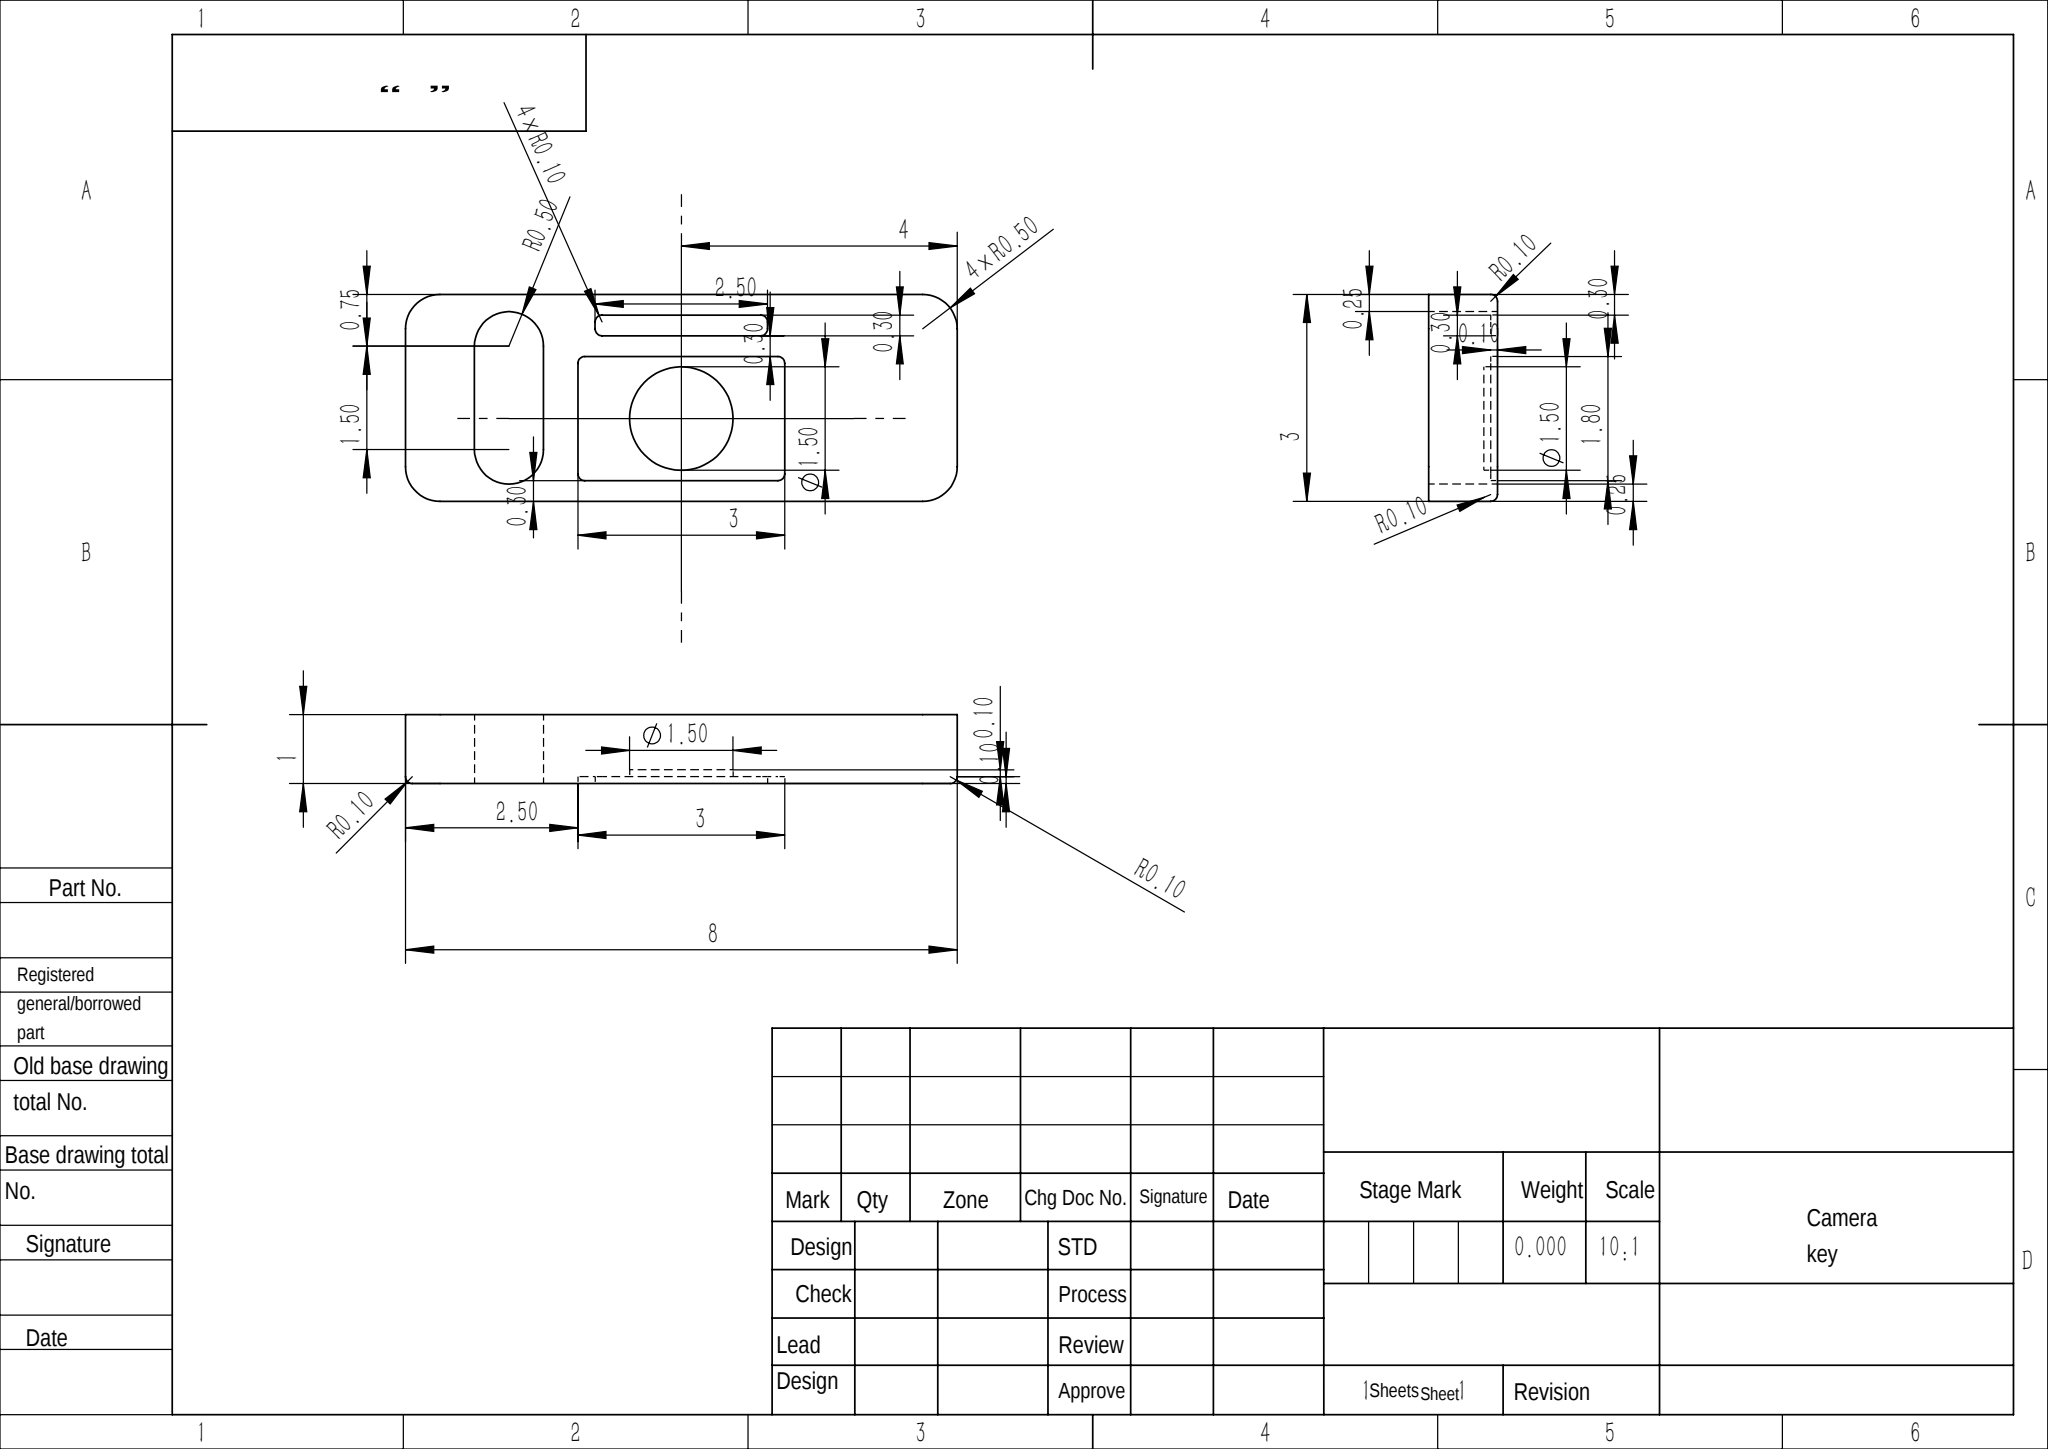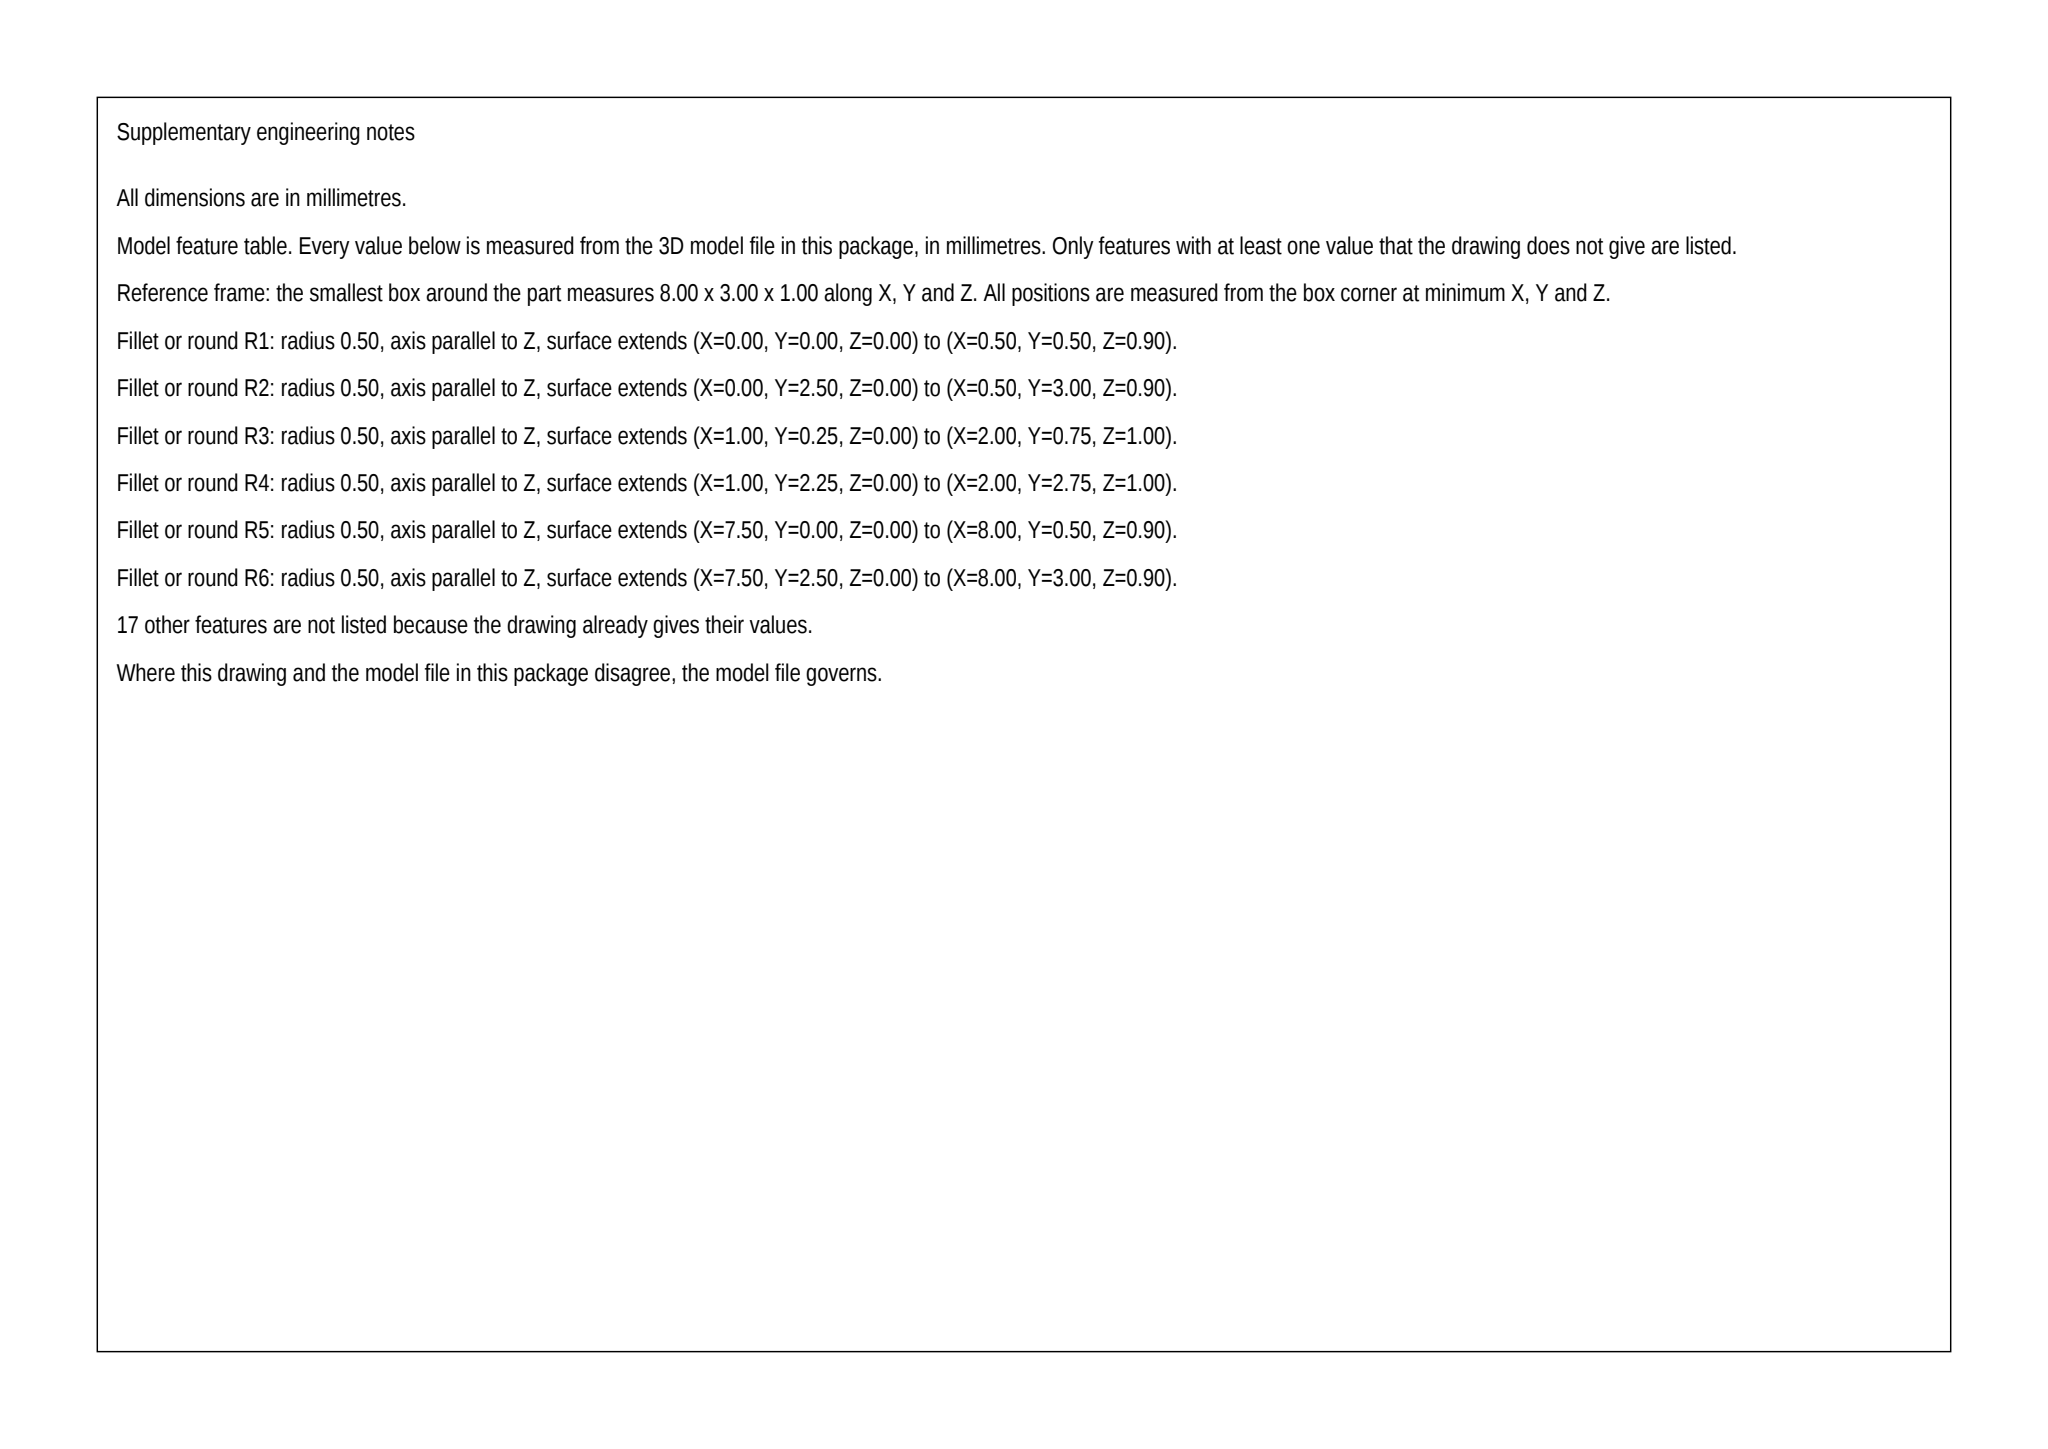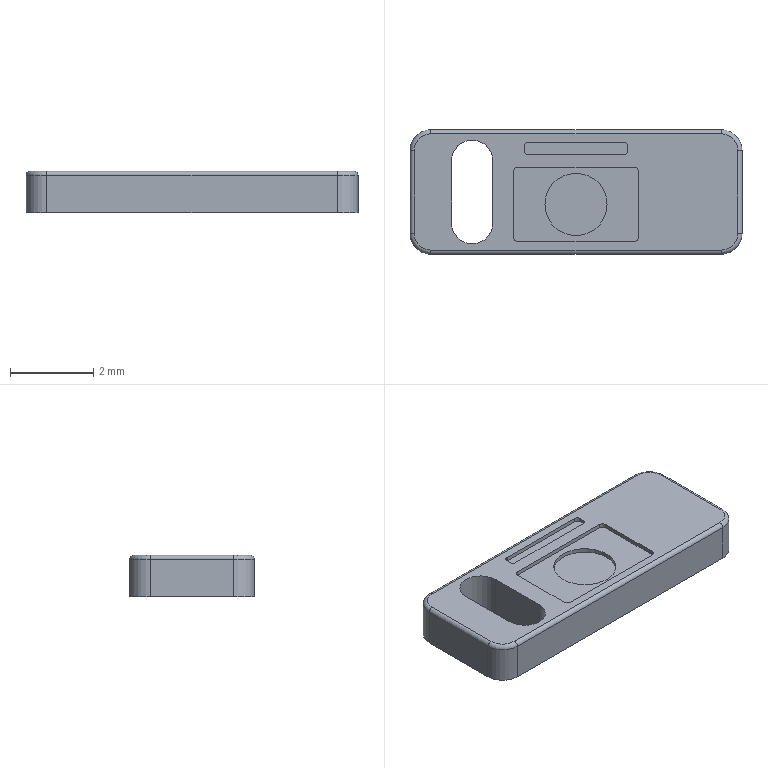Part | SolidWorks | mm | 1 solid | 43 faces | box 8 x 3 x 1 mm | volume 21 mm3 | cylinder 20 | plane 19 | torus 4 | commonest cylinder face diameters 0.2 x12 1 x6 1.5 x2
build123d program:
from build123d import *

# Parameters (mm, degrees)
SKETCH1_W           = 1
SKETCH1_H           = 3
BOSS_EXTRUDE1_DEPTH = 4
SKETCH2_3_W         = 2.5
SKETCH2_3_H         = 0.3
SKETCH2_3_W_2       = 3
SKETCH2_3_H_2       = 1.8
CUT_EXTRUDE1_DEPTH  = 0.1
SKETCH2_3_2_R       = 0.75
CUT_EXTRUDE3_DEPTH  = 0.2
FILLET1_R           = 0.5
FILLET2_R           = 0.1
FILLET3_R           = 0.1
CUT_EXTRUDE4_DEPTH  = 5


with BuildPart() as part:
    # Sketch1 → Boss-Extrude1 (new, symmetric)
    with BuildSketch(Plane(origin=(0, 0, 0), x_dir=(0, 0, -1), z_dir=(1, 0, 0))):
        Rectangle(SKETCH1_W, SKETCH1_H)
    extrude(amount=BOSS_EXTRUDE1_DEPTH, both=True)

    # Sketch2_3 → Cut-Extrude1 (cut)
    with BuildSketch(Plane.XY.offset(0.5)):
        with Locations((0, 1.05)):
            Rectangle(SKETCH2_3_W, SKETCH2_3_H)
        with Locations((0, -0.3)):
            Rectangle(SKETCH2_3_W_2, SKETCH2_3_H_2)
    extrude(amount=-CUT_EXTRUDE1_DEPTH, mode=Mode.SUBTRACT)

    # Sketch2_3 2 → Cut-Extrude3 (cut)
    with BuildSketch(Plane.XY.offset(0.5)):
        with Locations((0, -0.3)):
            Circle(SKETCH2_3_2_R)
    extrude(amount=-CUT_EXTRUDE3_DEPTH, mode=Mode.SUBTRACT)

    # Fillet1
    fillet1_edges = [part.edges().sort_by_distance(p)[0] for p in [
        (4, -1.5, 0),
        (-4, -1.5, 0),
        (-4, 1.5, 0),
        (4, 1.5, 0),
    ]]
    fillet(fillet1_edges, radius=FILLET1_R)

    # Fillet2
    fillet2_edges = [part.edges().sort_by_distance(p)[0] for p in [
        (0, -1.5, 0.5),
        (-4, 0, 0.5),
        (4, 0, 0.5),
        (0, 1.5, 0.5),
        (3.854, -1.354, 0.5),
        (3.854, 1.354, 0.5),
        (-3.854, 1.354, 0.5),
        (-3.854, -1.354, 0.5),
    ]]
    fillet(fillet2_edges, radius=FILLET2_R)

    # Fillet3
    fillet3_edges = [part.edges().sort_by_distance(p)[0] for p in [
        (1.25, 1.2, 0.45),
        (1.25, 0.9, 0.45),
        (-1.25, 0.9, 0.45),
        (-1.25, 1.2, 0.45),
        (-1.5, 0.6, 0.45),
        (1.5, 0.6, 0.45),
        (1.5, -1.2, 0.45),
        (-1.5, -1.2, 0.45),
    ]]
    fillet(fillet3_edges, radius=FILLET3_R)

    # Sketch4 → Cut-Extrude4 (cut, symmetric)
    with BuildSketch(Plane.XY):
        with BuildLine():
            Line((-3, -0.75), (-3, 0.75))
            ThreePointArc((-3, 0.75), (-2.5, 1.25), (-2, 0.75))
            Line((-2, 0.75), (-2, -0.75))
            ThreePointArc((-2, -0.75), (-2.5, -1.25), (-3, -0.75))
        make_face()
    extrude(amount=CUT_EXTRUDE4_DEPTH, both=True, mode=Mode.SUBTRACT)


solid = part.part